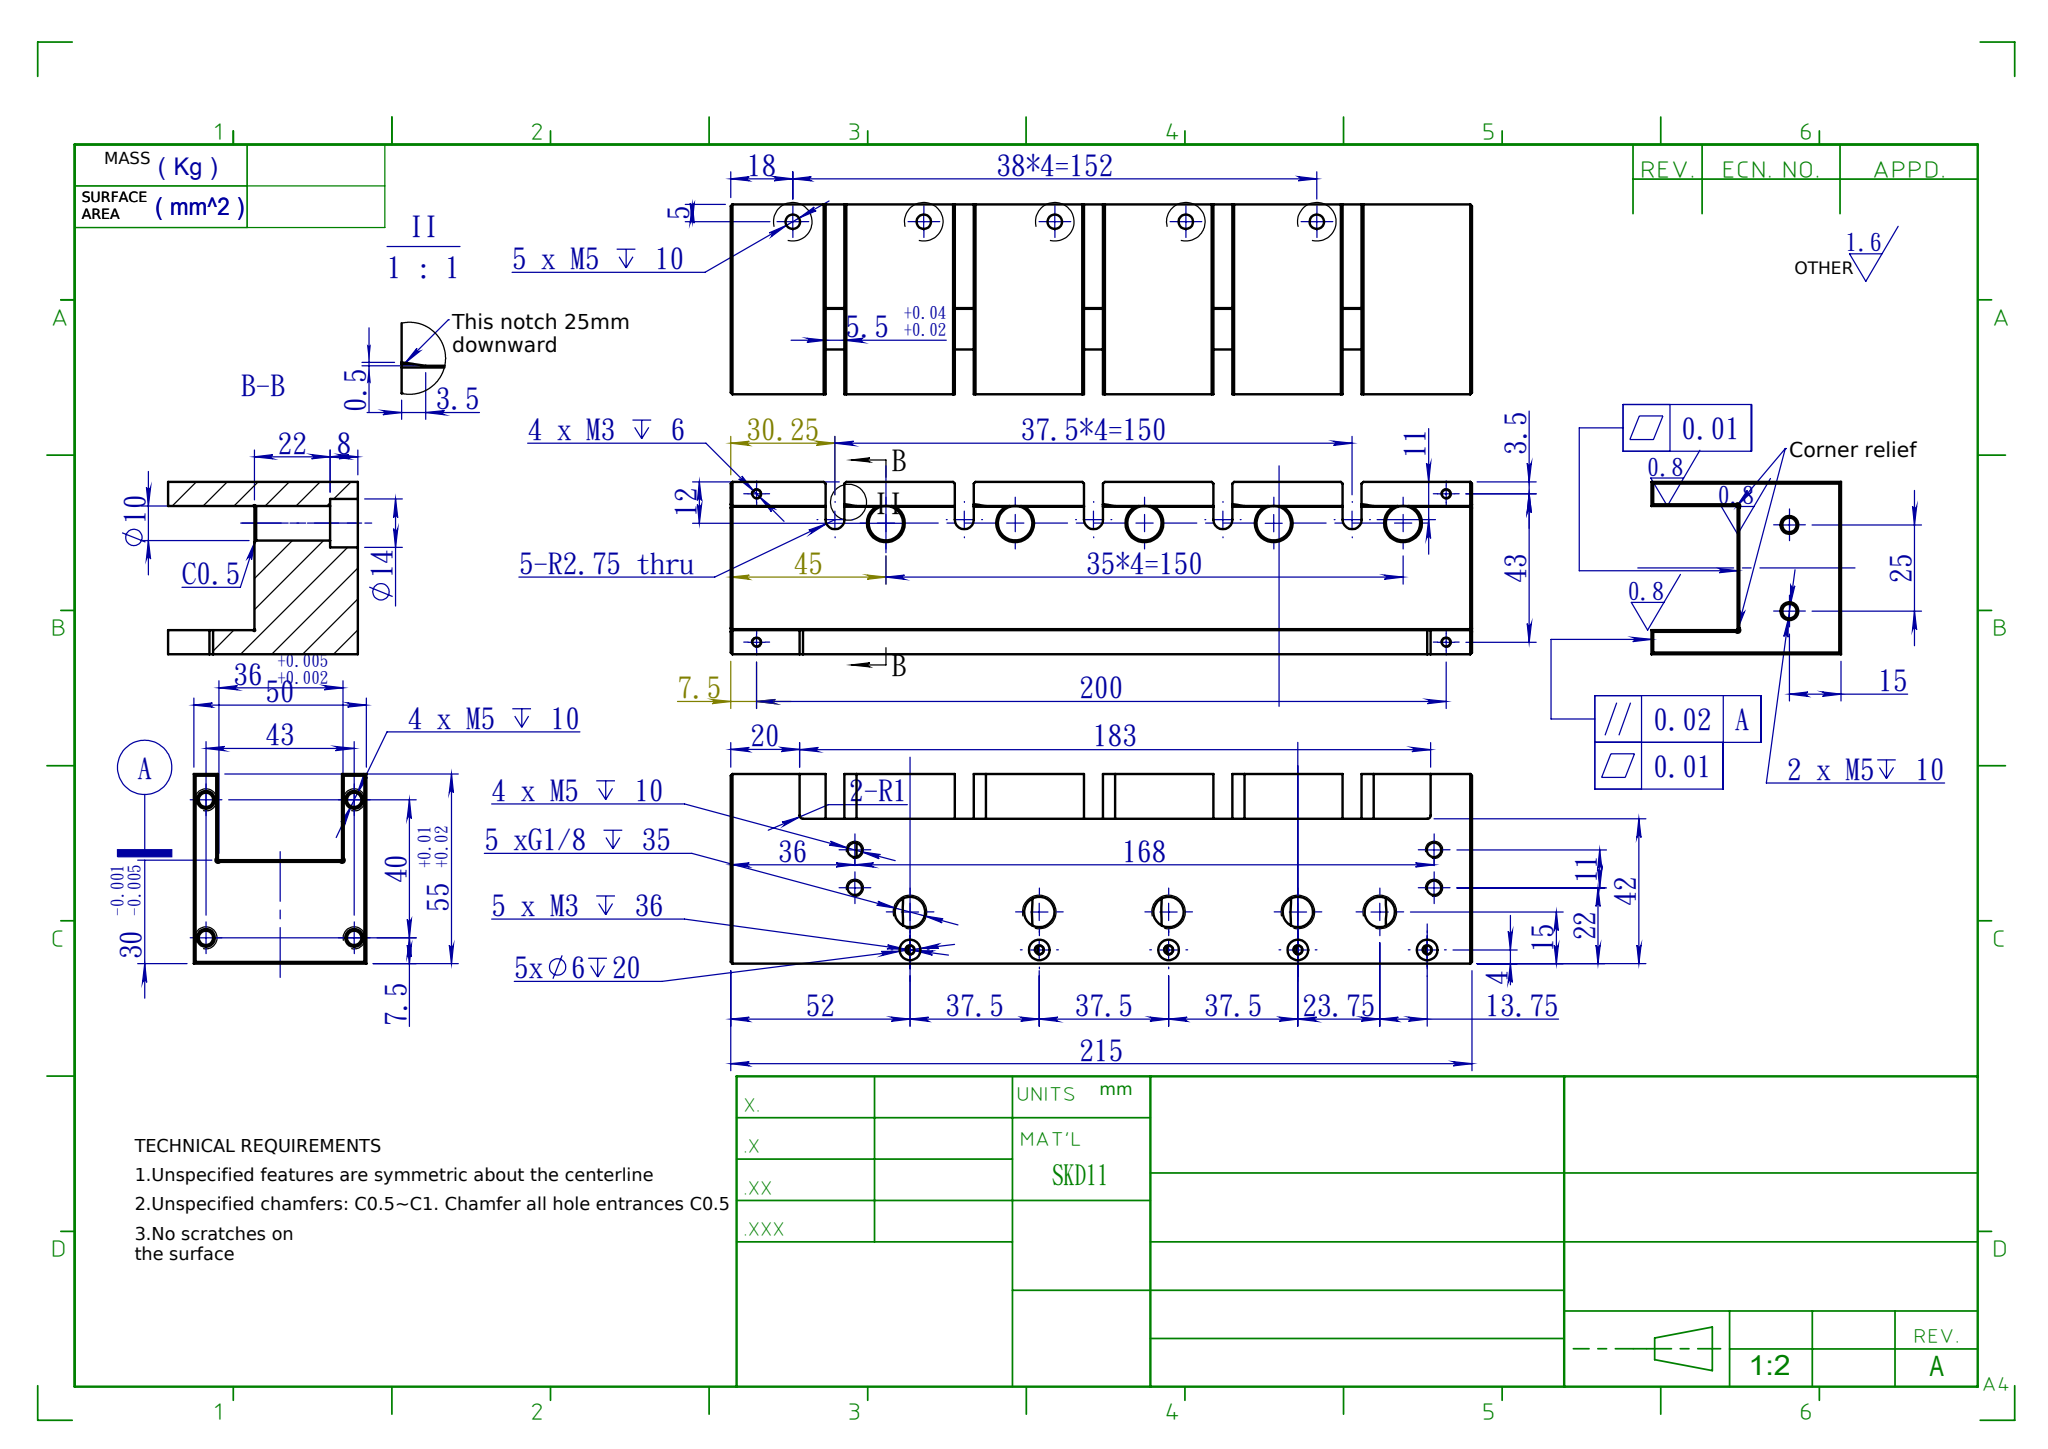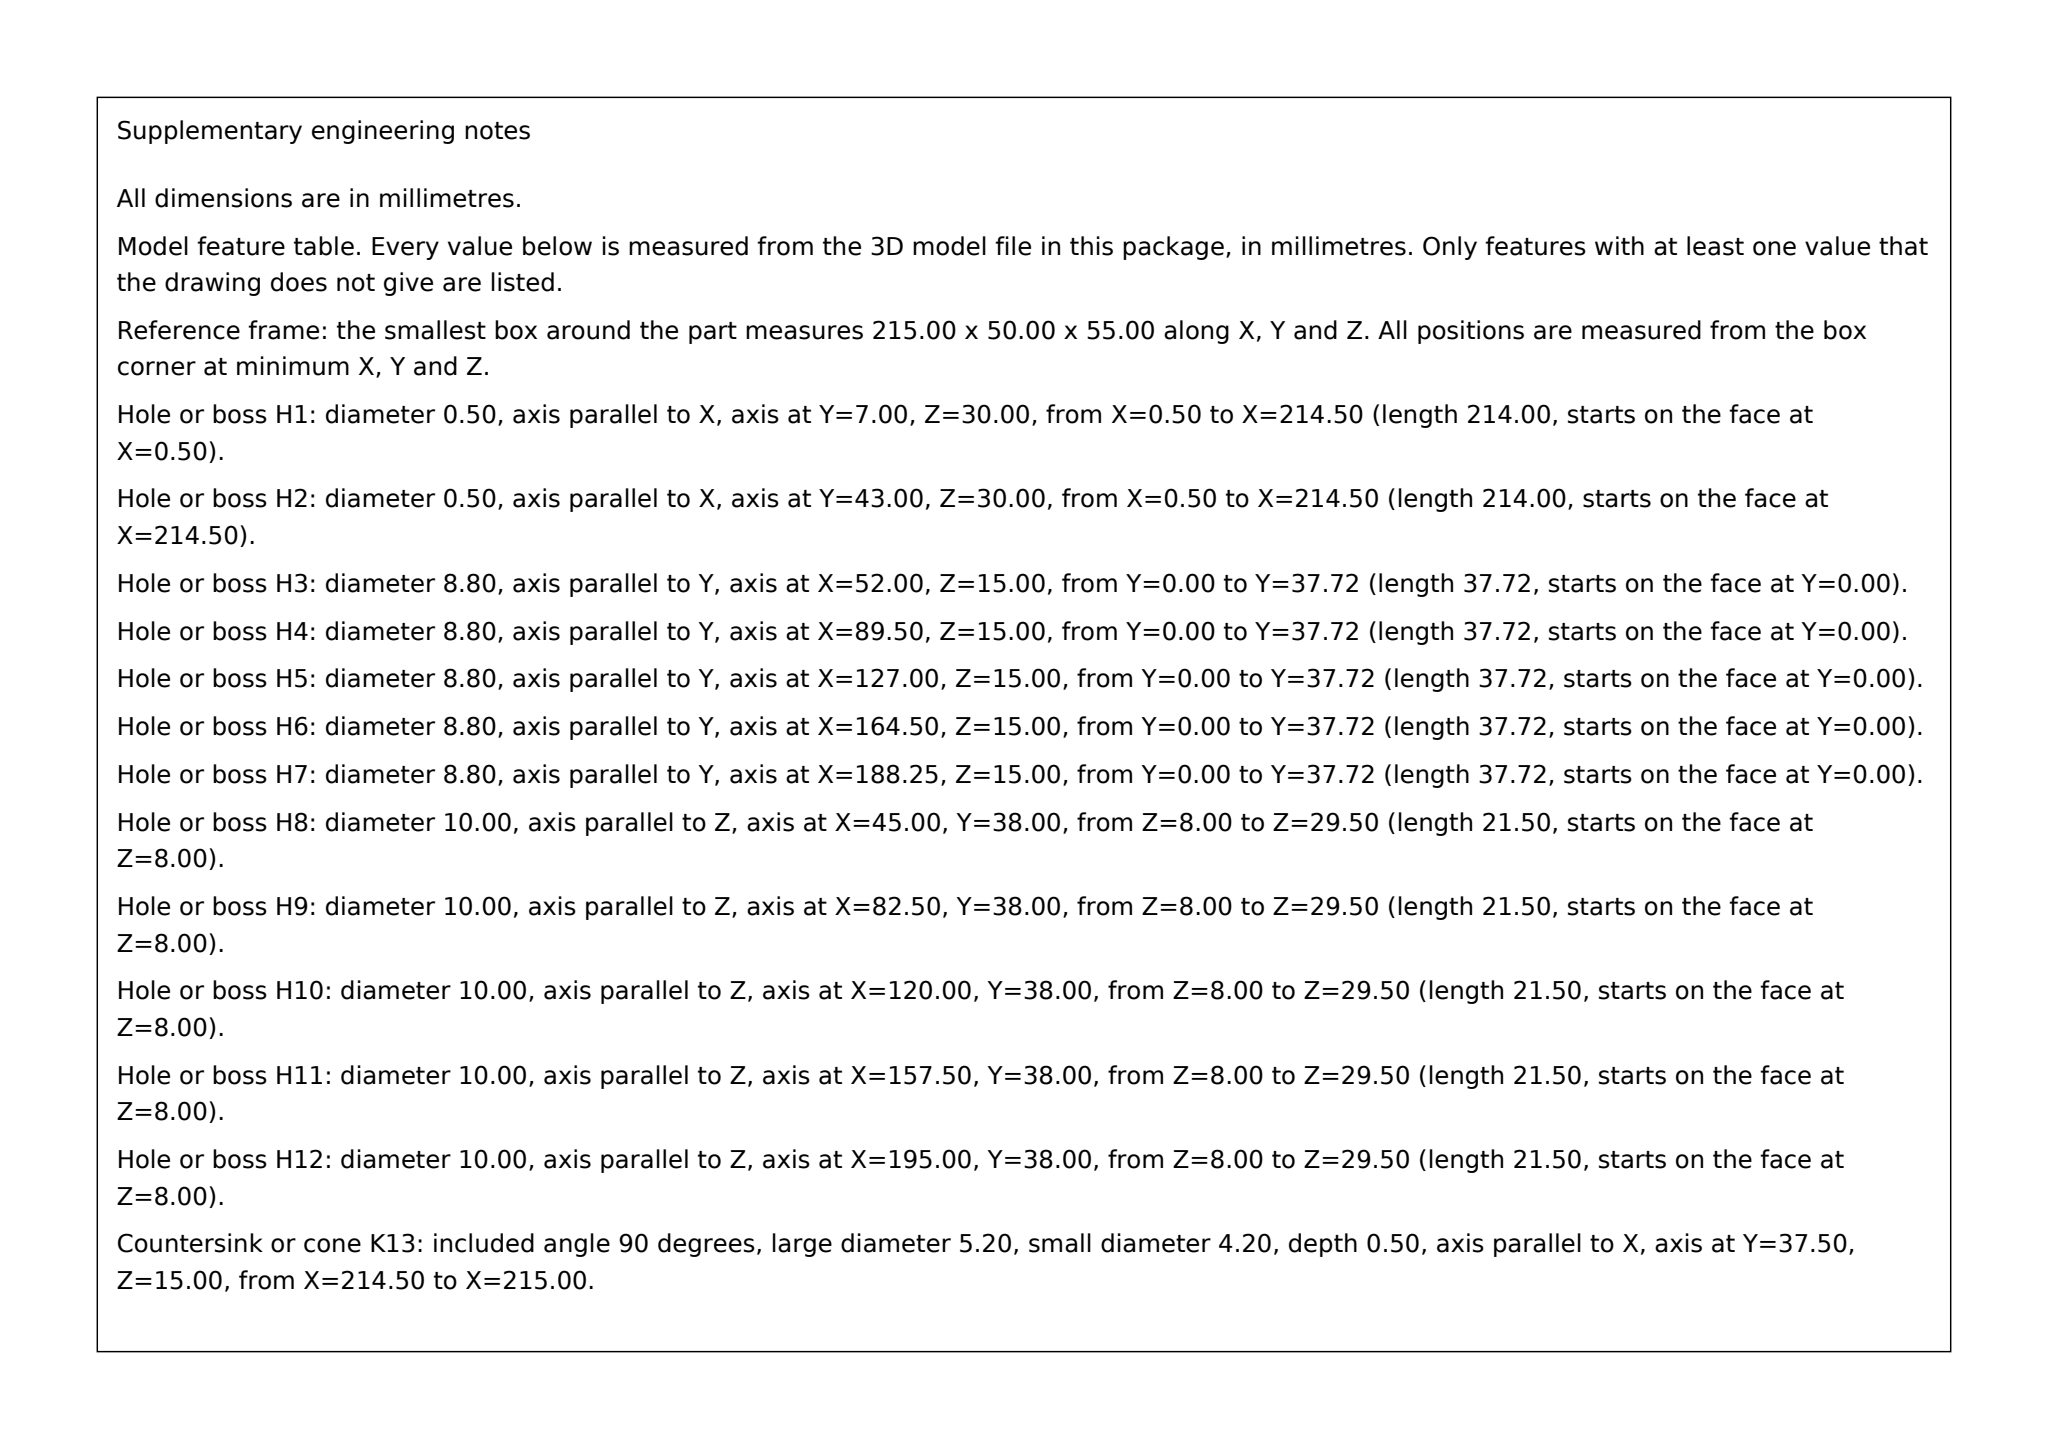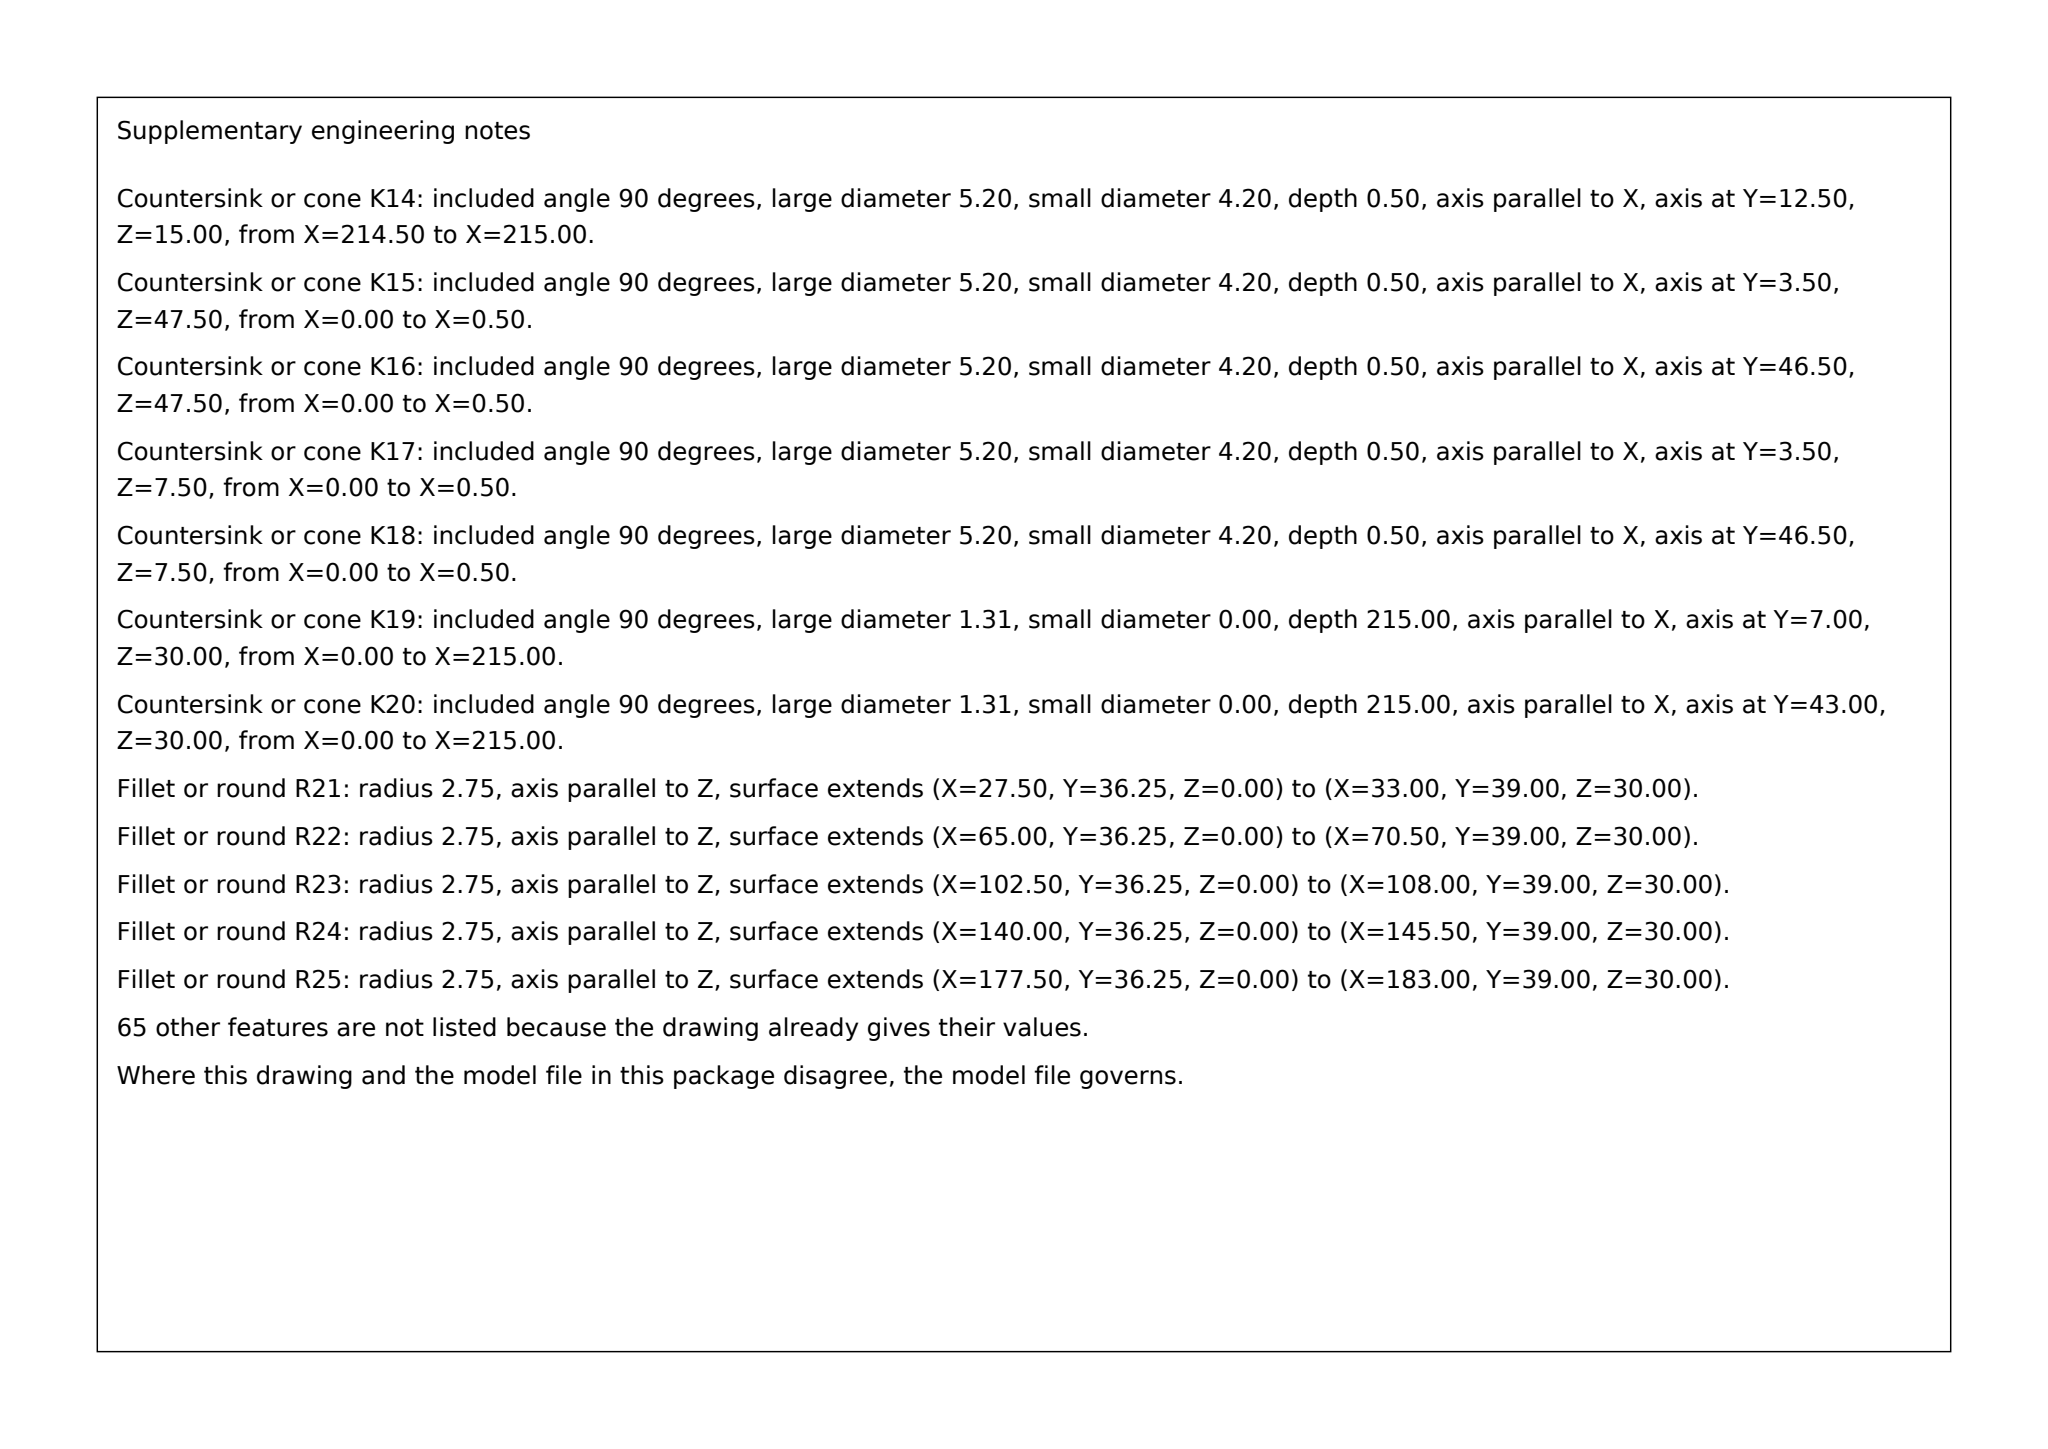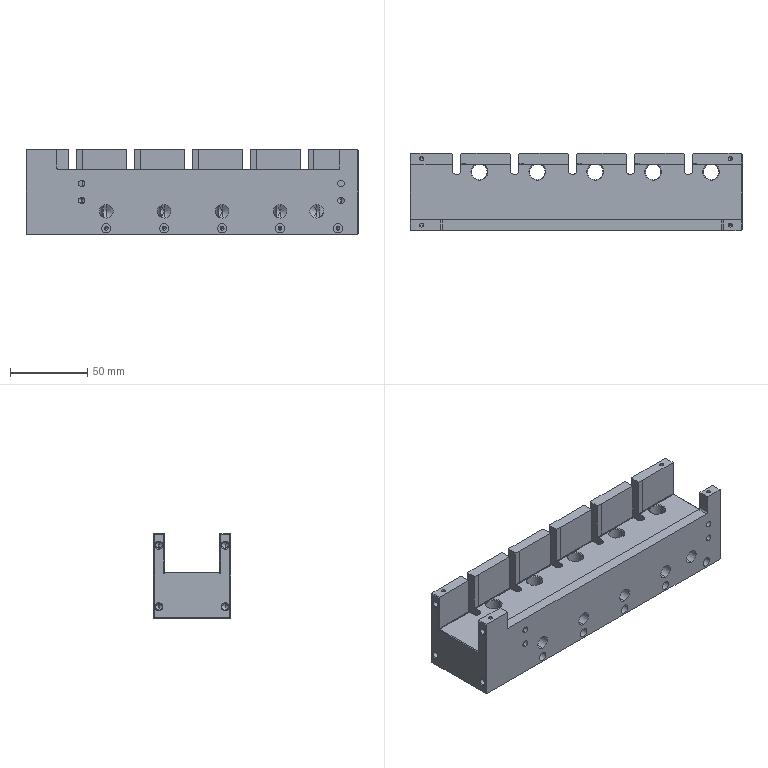Part | SolidWorks | mm | material SKD11 | 1 solid | 298 faces | box 215 x 50 x 55 mm | volume 332871 mm3 | cylinder 124 | plane 90 | cone 84 | commonest cylinder face diameters 4.2 x30 2.5 x28 0.5 x19 6 x10 8.8 x10 14 x10 10 x10 5.5 x5